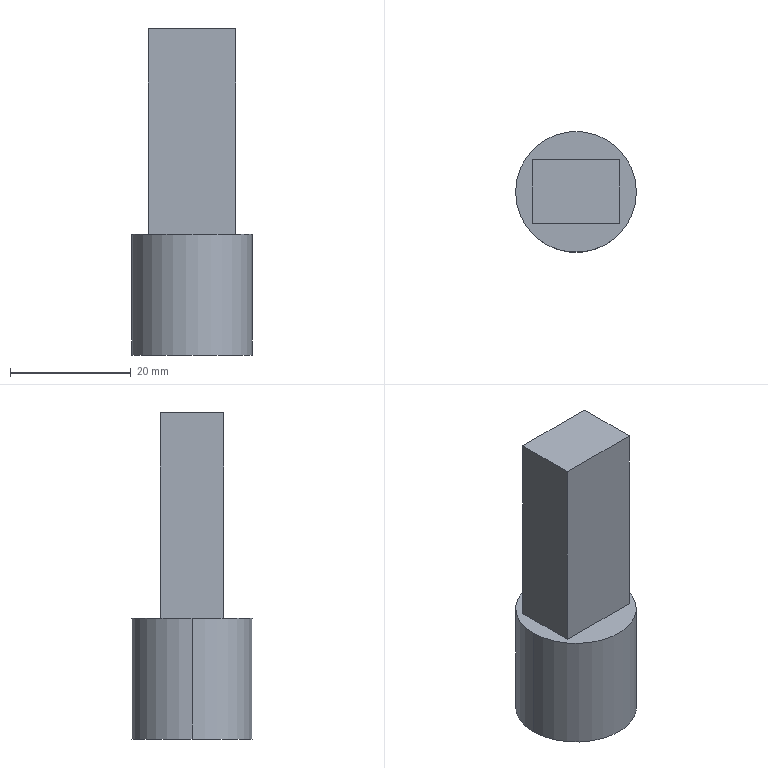Component | SolidWorks | CoilSleeveFixingRod-10 | 1 solid | 9 faces | box 20 x 20 x 54 mm | volume 11460 mm3 | plane 7 | cylinder 2 | commonest cylinder face diameters 20 x2 | material Plain Carbon Steel
build123d program:
from build123d import *

# Parameters (mm, degrees)
SKETCH1_W           = 10
SKETCH1_H           = 100
SKETCH2_W           = 14.5
SKETCH2_H           = 10.5
BOSS_EXTRUDE1_DEPTH = 34
MOVE_FACE1_BY       = 80


with BuildPart() as part:
    # Sketch1 → Revolve1 (revolve)
    with BuildSketch(Plane(origin=(0, 0, 0), x_dir=(1, 0, 0), z_dir=(0, 1, 0))):
        with Locations((5, -84)):
            Rectangle(SKETCH1_W, SKETCH1_H)
    revolve(axis=Axis((0, 0, 34), (0, 0, 1)))

    # Sketch2 → Boss-Extrude1 (add)
    with BuildSketch(Plane(origin=(0, 0, 34), x_dir=(-1, 0, 0), z_dir=(0, 0, -1))):
        Rectangle(SKETCH2_W, SKETCH2_H)
    extrude(amount=BOSS_EXTRUDE1_DEPTH)

    # Move Face1: a face moved inward by 80.0
    extrude(part.faces().sort_by_distance((0, 0, 134))[0], amount=MOVE_FACE1_BY, dir=(0, 0, -1), mode=Mode.SUBTRACT)


solid = part.part

# Placed as in the assembly
solid = solid.moved(Location((-864.885, 352.093, 1139.102), (180, 0, 0)))
STEP:
#1=COLOUR_RGB('',0.7922,0.8196,0.9333);
#2=FILL_AREA_STYLE_COLOUR('',#1);
#3=FILL_AREA_STYLE('',(#2));
#4=SURFACE_STYLE_FILL_AREA(#3);
#5=SURFACE_SIDE_STYLE('',(#4));
#6=SURFACE_STYLE_USAGE(.BOTH.,#5);
#7=PRESENTATION_STYLE_ASSIGNMENT((#6));
#8=CARTESIAN_POINT('',(-33.657,13.862,43.508));
#9=VERTEX_POINT('',#8);
#10=CARTESIAN_POINT('',(-34.444,13.862,43.508));
#11=VERTEX_POINT('',#10);
#12=CARTESIAN_POINT('',(-34.051,13.862,43.508));
#13=DIRECTION('',(-0.,0.,-1.));
#14=DIRECTION('',(1.,0.,0.));
#15=AXIS2_PLACEMENT_3D('',#12,#13,#14);
#16=CIRCLE('',#15,0.3937);
#17=EDGE_CURVE('',#9,#11,#16,.T.);
#18=ORIENTED_EDGE('',*,*,#17,.T.);
#19=CARTESIAN_POINT('',(-34.444,13.862,42.721));
#20=VERTEX_POINT('',#19);
#21=CARTESIAN_POINT('',(-34.444,13.862,43.508));
#22=DIRECTION('',(-0.,0.,-1.));
#23=VECTOR('',#22,39.37);
#24=LINE('',#21,#23);
#25=EDGE_CURVE('',#11,#20,#24,.T.);
#26=ORIENTED_EDGE('',*,*,#25,.T.);
#27=CARTESIAN_POINT('',(-33.657,13.862,42.721));
#28=VERTEX_POINT('',#27);
#29=CARTESIAN_POINT('',(-34.051,13.862,42.721));
#30=DIRECTION('',(-0.,0.,-1.));
#31=DIRECTION('',(1.,0.,0.));
#32=AXIS2_PLACEMENT_3D('',#29,#30,#31);
#33=CIRCLE('',#32,0.3937);
#34=EDGE_CURVE('',#28,#20,#33,.T.);
#35=ORIENTED_EDGE('',*,*,#34,.F.);
#36=CARTESIAN_POINT('',(-33.657,13.862,43.508));
#37=DIRECTION('',(-0.,0.,-1.));
#38=VECTOR('',#37,39.37);
#39=LINE('',#36,#38);
#40=EDGE_CURVE('',#9,#28,#39,.T.);
#41=ORIENTED_EDGE('',*,*,#40,.F.);
#42=EDGE_LOOP('',(#18,#26,#35,#41));
#43=FACE_OUTER_BOUND('',#42,.T.);
#44=CARTESIAN_POINT('',(-34.051,13.862,43.508));
#45=DIRECTION('',(-0.,0.,-1.));
#46=DIRECTION('',(1.,0.,0.));
#47=AXIS2_PLACEMENT_3D('',#44,#45,#46);
#48=CYLINDRICAL_SURFACE('',#47,0.3937);
#49=ADVANCED_FACE('',(#43),#48,.T.);
#50=ORIENTED_EDGE('',*,*,#17,.F.);
#51=CARTESIAN_POINT('',(-34.051,13.862,43.508));
#52=DIRECTION('',(-0.,0.,-1.));
#53=DIRECTION('',(1.,0.,0.));
#54=AXIS2_PLACEMENT_3D('',#51,#52,#53);
#55=CIRCLE('',#54,0.3937);
#56=EDGE_CURVE('',#11,#9,#55,.T.);
#57=ORIENTED_EDGE('',*,*,#56,.F.);
#58=EDGE_LOOP('',(#50,#57));
#59=FACE_OUTER_BOUND('',#58,.T.);
#60=CARTESIAN_POINT('',(-33.765,14.069,43.508));
#61=VERTEX_POINT('',#60);
#62=CARTESIAN_POINT('',(-34.336,14.069,43.508));
#63=VERTEX_POINT('',#62);
#64=CARTESIAN_POINT('',(-34.336,14.069,43.508));
#65=DIRECTION('',(-1.,-0.,0.));
#66=VECTOR('',#65,39.37);
#67=LINE('',#64,#66);
#68=EDGE_CURVE('',#61,#63,#67,.T.);
#69=ORIENTED_EDGE('',*,*,#68,.F.);
#70=CARTESIAN_POINT('',(-33.765,13.655,43.508));
#71=VERTEX_POINT('',#70);
#72=CARTESIAN_POINT('',(-33.765,14.069,43.508));
#73=DIRECTION('',(0.,1.,0.));
#74=VECTOR('',#73,39.37);
#75=LINE('',#72,#74);
#76=EDGE_CURVE('',#71,#61,#75,.T.);
#77=ORIENTED_EDGE('',*,*,#76,.F.);
#78=CARTESIAN_POINT('',(-34.336,13.655,43.508));
#79=VERTEX_POINT('',#78);
#80=CARTESIAN_POINT('',(-33.765,13.655,43.508));
#81=DIRECTION('',(1.,0.,-0.));
#82=VECTOR('',#81,39.37);
#83=LINE('',#80,#82);
#84=EDGE_CURVE('',#79,#71,#83,.T.);
#85=ORIENTED_EDGE('',*,*,#84,.F.);
#86=CARTESIAN_POINT('',(-34.336,13.655,43.508));
#87=DIRECTION('',(0.,-1.,-0.));
#88=VECTOR('',#87,39.37);
#89=LINE('',#86,#88);
#90=EDGE_CURVE('',#63,#79,#89,.T.);
#91=ORIENTED_EDGE('',*,*,#90,.F.);
#92=EDGE_LOOP('',(#69,#77,#85,#91));
#93=FACE_BOUND('',#92,.T.);
#94=CARTESIAN_POINT('',(-33.657,13.862,43.508));
#95=DIRECTION('',(0.,-0.,1.));
#96=DIRECTION('',(-1.,-0.,0.));
#97=AXIS2_PLACEMENT_3D('',#94,#95,#96);
#98=PLANE('',#97);
#99=ADVANCED_FACE('',(#59,#93),#98,.T.);
#100=ORIENTED_EDGE('',*,*,#25,.F.);
#101=ORIENTED_EDGE('',*,*,#56,.T.);
#102=ORIENTED_EDGE('',*,*,#40,.T.);
#103=CARTESIAN_POINT('',(-34.051,13.862,42.721));
#104=DIRECTION('',(-0.,0.,-1.));
#105=DIRECTION('',(1.,0.,0.));
#106=AXIS2_PLACEMENT_3D('',#103,#104,#105);
#107=CIRCLE('',#106,0.3937);
#108=EDGE_CURVE('',#20,#28,#107,.T.);
#109=ORIENTED_EDGE('',*,*,#108,.F.);
#110=EDGE_LOOP('',(#100,#101,#102,#109));
#111=FACE_OUTER_BOUND('',#110,.T.);
#112=CARTESIAN_POINT('',(-34.051,13.862,43.508));
#113=DIRECTION('',(-0.,0.,-1.));
#114=DIRECTION('',(1.,0.,0.));
#115=AXIS2_PLACEMENT_3D('',#112,#113,#114);
#116=CYLINDRICAL_SURFACE('',#115,0.3937);
#117=ADVANCED_FACE('',(#111),#116,.T.);
#118=ORIENTED_EDGE('',*,*,#34,.T.);
#119=ORIENTED_EDGE('',*,*,#108,.T.);
#120=EDGE_LOOP('',(#118,#119));
#121=FACE_OUTER_BOUND('',#120,.T.);
#122=CARTESIAN_POINT('',(-34.051,13.862,42.721));
#123=DIRECTION('',(-0.,0.,-1.));
#124=DIRECTION('',(1.,0.,-0.));
#125=AXIS2_PLACEMENT_3D('',#122,#123,#124);
#126=PLANE('',#125);
#127=ADVANCED_FACE('',(#121),#126,.T.);
#128=ORIENTED_EDGE('',*,*,#76,.T.);
#129=CARTESIAN_POINT('',(-33.765,14.069,44.847));
#130=VERTEX_POINT('',#129);
#131=CARTESIAN_POINT('',(-33.765,14.069,44.847));
#132=DIRECTION('',(-0.,0.,-1.));
#133=VECTOR('',#132,39.37);
#134=LINE('',#131,#133);
#135=EDGE_CURVE('',#130,#61,#134,.T.);
#136=ORIENTED_EDGE('',*,*,#135,.F.);
#137=CARTESIAN_POINT('',(-33.765,13.655,44.847));
#138=VERTEX_POINT('',#137);
#139=CARTESIAN_POINT('',(-33.765,14.069,44.847));
#140=DIRECTION('',(0.,1.,0.));
#141=VECTOR('',#140,39.37);
#142=LINE('',#139,#141);
#143=EDGE_CURVE('',#138,#130,#142,.T.);
#144=ORIENTED_EDGE('',*,*,#143,.F.);
#145=CARTESIAN_POINT('',(-33.765,13.655,44.847));
#146=DIRECTION('',(-0.,0.,-1.));
#147=VECTOR('',#146,39.37);
#148=LINE('',#145,#147);
#149=EDGE_CURVE('',#138,#71,#148,.T.);
#150=ORIENTED_EDGE('',*,*,#149,.T.);
#151=EDGE_LOOP('',(#128,#136,#144,#150));
#152=FACE_OUTER_BOUND('',#151,.T.);
#153=CARTESIAN_POINT('',(-33.765,14.069,44.847));
#154=DIRECTION('',(-1.,-0.,0.));
#155=DIRECTION('',(-0.,0.,-1.));
#156=AXIS2_PLACEMENT_3D('',#153,#154,#155);
#157=PLANE('',#156);
#158=ADVANCED_FACE('',(#152),#157,.F.);
#159=ORIENTED_EDGE('',*,*,#68,.T.);
#160=CARTESIAN_POINT('',(-34.336,14.069,44.847));
#161=VERTEX_POINT('',#160);
#162=CARTESIAN_POINT('',(-34.336,14.069,44.847));
#163=DIRECTION('',(-0.,0.,-1.));
#164=VECTOR('',#163,39.37);
#165=LINE('',#162,#164);
#166=EDGE_CURVE('',#161,#63,#165,.T.);
#167=ORIENTED_EDGE('',*,*,#166,.F.);
#168=CARTESIAN_POINT('',(-34.336,14.069,44.847));
#169=DIRECTION('',(-1.,-0.,0.));
#170=VECTOR('',#169,39.37);
#171=LINE('',#168,#170);
#172=EDGE_CURVE('',#130,#161,#171,.T.);
#173=ORIENTED_EDGE('',*,*,#172,.F.);
#174=ORIENTED_EDGE('',*,*,#135,.T.);
#175=EDGE_LOOP('',(#159,#167,#173,#174));
#176=FACE_OUTER_BOUND('',#175,.T.);
#177=CARTESIAN_POINT('',(-34.336,14.069,44.847));
#178=DIRECTION('',(-0.,-1.,-0.));
#179=DIRECTION('',(-0.,0.,-1.));
#180=AXIS2_PLACEMENT_3D('',#177,#178,#179);
#181=PLANE('',#180);
#182=ADVANCED_FACE('',(#176),#181,.F.);
#183=ORIENTED_EDGE('',*,*,#90,.T.);
#184=CARTESIAN_POINT('',(-34.336,13.655,44.847));
#185=VERTEX_POINT('',#184);
#186=CARTESIAN_POINT('',(-34.336,13.655,44.847));
#187=DIRECTION('',(-0.,0.,-1.));
#188=VECTOR('',#187,39.37);
#189=LINE('',#186,#188);
#190=EDGE_CURVE('',#185,#79,#189,.T.);
#191=ORIENTED_EDGE('',*,*,#190,.F.);
#192=CARTESIAN_POINT('',(-34.336,13.655,44.847));
#193=DIRECTION('',(0.,-1.,-0.));
#194=VECTOR('',#193,39.37);
#195=LINE('',#192,#194);
#196=EDGE_CURVE('',#161,#185,#195,.T.);
#197=ORIENTED_EDGE('',*,*,#196,.F.);
#198=ORIENTED_EDGE('',*,*,#166,.T.);
#199=EDGE_LOOP('',(#183,#191,#197,#198));
#200=FACE_OUTER_BOUND('',#199,.T.);
#201=CARTESIAN_POINT('',(-34.336,13.655,44.847));
#202=DIRECTION('',(1.,0.,-0.));
#203=DIRECTION('',(0.,-0.,1.));
#204=AXIS2_PLACEMENT_3D('',#201,#202,#203);
#205=PLANE('',#204);
#206=ADVANCED_FACE('',(#200),#205,.F.);
#207=ORIENTED_EDGE('',*,*,#84,.T.);
#208=ORIENTED_EDGE('',*,*,#149,.F.);
#209=CARTESIAN_POINT('',(-33.765,13.655,44.847));
#210=DIRECTION('',(1.,0.,-0.));
#211=VECTOR('',#210,39.37);
#212=LINE('',#209,#211);
#213=EDGE_CURVE('',#185,#138,#212,.T.);
#214=ORIENTED_EDGE('',*,*,#213,.F.);
#215=ORIENTED_EDGE('',*,*,#190,.T.);
#216=EDGE_LOOP('',(#207,#208,#214,#215));
#217=FACE_OUTER_BOUND('',#216,.T.);
#218=CARTESIAN_POINT('',(-33.765,13.655,44.847));
#219=DIRECTION('',(0.,1.,0.));
#220=DIRECTION('',(0.,-0.,1.));
#221=AXIS2_PLACEMENT_3D('',#218,#219,#220);
#222=PLANE('',#221);
#223=ADVANCED_FACE('',(#217),#222,.F.);
#224=ORIENTED_EDGE('',*,*,#143,.T.);
#225=ORIENTED_EDGE('',*,*,#172,.T.);
#226=ORIENTED_EDGE('',*,*,#196,.T.);
#227=ORIENTED_EDGE('',*,*,#213,.T.);
#228=EDGE_LOOP('',(#224,#225,#226,#227));
#229=FACE_OUTER_BOUND('',#228,.T.);
#230=CARTESIAN_POINT('',(-34.051,13.862,44.847));
#231=DIRECTION('',(-0.,0.,-1.));
#232=DIRECTION('',(1.,0.,-0.));
#233=AXIS2_PLACEMENT_3D('',#230,#231,#232);
#234=PLANE('',#233);
#235=ADVANCED_FACE('',(#229),#234,.F.);
#236=CLOSED_SHELL('',(#49,#99,#117,#127,#158,#182,#206,#223,#235));
#237=MANIFOLD_SOLID_BREP('',#236);
#238=STYLED_ITEM('',(#7),#237);
#239=PRESENTATION_LAYER_ASSIGNMENT('','',(#238));
#240=CARTESIAN_POINT('',(0.,0.,0.));
#241=DIRECTION('',(0.,0.,1.));
#242=DIRECTION('',(1.,0.,0.));
#243=AXIS2_PLACEMENT_3D('',#240,#241,#242);
#244=(LENGTH_UNIT()NAMED_UNIT(*)SI_UNIT($,.METRE.));
#245=LENGTH_MEASURE_WITH_UNIT(LENGTH_MEASURE(0.0254),#244);
#246=DIMENSIONAL_EXPONENTS(1.,0.,0.,0.,0.,0.,0.);
#247=(CONVERSION_BASED_UNIT('',#245)LENGTH_UNIT()NAMED_UNIT(#246));
#248=UNCERTAINTY_MEASURE_WITH_UNIT(LENGTH_MEASURE(0.00001),#247,'','');
#249=(NAMED_UNIT(*)PLANE_ANGLE_UNIT()SI_UNIT($,.RADIAN.));
#250=(NAMED_UNIT(*)SI_UNIT($,.STERADIAN.)SOLID_ANGLE_UNIT());
#251=(GEOMETRIC_REPRESENTATION_CONTEXT(3)GLOBAL_UNCERTAINTY_ASSIGNED_CONTEXT((#248))GLOBAL_UNIT_ASSIGNED_CONTEXT((#247,#249,#250))REPRESENTATION_CONTEXT('',''));
#252=ADVANCED_BREP_SHAPE_REPRESENTATION('',(#237,#243),#251);
#253=(LENGTH_UNIT()NAMED_UNIT(*)SI_UNIT($,.METRE.));
#254=LENGTH_MEASURE_WITH_UNIT(LENGTH_MEASURE(0.0254),#253);
#255=DIMENSIONAL_EXPONENTS(1.,0.,0.,0.,0.,0.,0.);
#256=(CONVERSION_BASED_UNIT('',#254)LENGTH_UNIT()NAMED_UNIT(#255));
#257=UNCERTAINTY_MEASURE_WITH_UNIT(LENGTH_MEASURE(0.00001),#256,'','');
#258=(NAMED_UNIT(*)PLANE_ANGLE_UNIT()SI_UNIT($,.RADIAN.));
#259=(NAMED_UNIT(*)SI_UNIT($,.STERADIAN.)SOLID_ANGLE_UNIT());
#260=(GEOMETRIC_REPRESENTATION_CONTEXT(3)GLOBAL_UNCERTAINTY_ASSIGNED_CONTEXT((#257))GLOBAL_UNIT_ASSIGNED_CONTEXT((#256,#258,#259))REPRESENTATION_CONTEXT('',''));
#261=MECHANICAL_DESIGN_GEOMETRIC_PRESENTATION_REPRESENTATION('',(#238),#260);